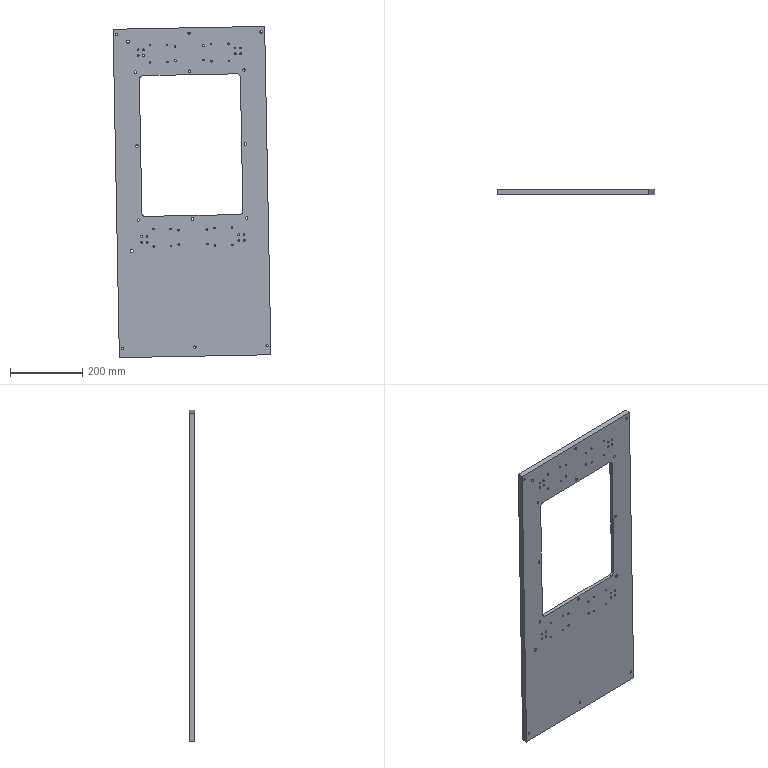Component | SolidWorks | 09Panel2-1 | 1 solid | 224 faces | box 437.25 x 15 x 917.83 mm | volume 3859009 mm3 | cylinder 134 | cone 68 | plane 22 | commonest cylinder face diameters 5 x48 4.2 x32 6.8 x16 11 x12 6.6 x12 8.5 x4 30 x4 20 x4 | material A3 Steel
build123d program:
from build123d import *

# Parameters (mm, degrees)
SKETCH1_W                                          = 900
SKETCH1_H                                          = 420
BOSS_EXTRUDE1_DEPTH                                = 7.5
HOLE_SIZE_ACCORDING_TO_TYPE_1_OF_HEXAG_D           = 6.6
HOLE_SIZE_ACCORDING_TO_TYPE_1_OF_HEXAG_CBORE_D     = 11
HOLE_SIZE_ACCORDING_TO_TYPE_1_OF_HEXAG_CBORE_DEPTH = 8
M10_TAPPED_HOLE1_D                                 = 8.5
M10_TAPPED_HOLE1_CSINK_D                           = 10.05
M10_TAPPED_HOLE1_CSINK_ANGLE                       = 90
CUT_EXTRUDE1_DEPTH                                 = 6
CUT_EXTRUDE2_DEPTH                                 = 497.67
M8_TAPPED_HOLE1_D                                  = 6.8
M8_TAPPED_HOLE1_CSINK_D                            = 8.05
M8_TAPPED_HOLE1_CSINK_ANGLE                        = 90
SKETCH12_R                                         = 20
CUT_EXTRUDE3_DEPTH                                 = 497.815
M6_TAPPED_HOLE1_D                                  = 5
M6_TAPPED_HOLE1_CSINK_D                            = 6.05
M6_TAPPED_HOLE1_CSINK_ANGLE                        = 90
LPATTERN1_COUNT                                    = 2
LPATTERN1_PITCH                                    = 510
M5_TAPPED_HOLE1_D                                  = 4.2
M5_TAPPED_HOLE1_CSINK_D                            = 5.05
M5_TAPPED_HOLE1_CSINK_ANGLE                        = 90
LPATTERN3_COUNT                                    = 2
LPATTERN3_PITCH                                    = 170
LPATTERN3_COUNT_DIR2                               = 2
LPATTERN3_PITCH_DIR2                               = 510
CUT_EXTRUDE4_REACH                                 = 617.594
SKETCH20_R                                         = 6.062
M6_TAPPED_HOLE2_D                                  = 5
MIRROR2_COPY_1_D                                   = 5
SKETCH24_W                                         = 15
SKETCH24_H                                         = 420
BOSS_EXTRUDE2_DEPTH                                = 10
BOSS_EXTRUDE3_START                                = -15
SKETCH25_R                                         = 20
BOSS_EXTRUDE3_DEPTH                                = 15


with BuildPart() as part:
    # Sketch1 → Boss-Extrude1 (new, symmetric)
    with BuildSketch(Plane.XY):
        Rectangle(SKETCH1_W, SKETCH1_H)
    extrude(amount=BOSS_EXTRUDE1_DEPTH, both=True)

    # Hole Size _According to_ Type 1 of Hexag (through all)
    with Locations(Plane(origin=(-435, 200, 7.5), x_dir=(1, 0, 0), z_dir=(0, 0, 1))):
        with Locations((0, 0), (870, 0), (870, -400), (0, -400), (0, -200), (870, -200)):
            CounterBoreHole(HOLE_SIZE_ACCORDING_TO_TYPE_1_OF_HEXAG_D / 2, HOLE_SIZE_ACCORDING_TO_TYPE_1_OF_HEXAG_CBORE_D / 2, HOLE_SIZE_ACCORDING_TO_TYPE_1_OF_HEXAG_CBORE_DEPTH)

    # M10 Tapped Hole1 (through all)
    with Locations(Plane(origin=(-165, -170, 7.5), x_dir=(1, 0, 0), z_dir=(0, 0, 1))):
        with Locations((0, 0), (580, 0)):
            CounterSinkHole(M10_TAPPED_HOLE1_D / 2, M10_TAPPED_HOLE1_CSINK_D / 2, counter_sink_angle=M10_TAPPED_HOLE1_CSINK_ANGLE)

    # Sketch8 → Cut-Extrude1 (cut)
    with BuildSketch(Plane.XY.offset(7.5)):
        with BuildLine():
            Line((-80, -165), (330, -165))
            ThreePointArc((330, -165), (340.607, -160.607), (345, -150))
            Line((345, -150), (345, 150))
            ThreePointArc((345, 150), (340.607, 160.607), (330, 165))
            Line((330, 165), (-80, 165))
            ThreePointArc((-80, 165), (-90.607, 160.607), (-95, 150))
            Line((-95, 150), (-95, -150))
            ThreePointArc((-95, -150), (-90.607, -160.607), (-80, -165))
        make_face()
    extrude(amount=-CUT_EXTRUDE1_DEPTH, mode=Mode.SUBTRACT)

    # Sketch9 → Cut-Extrude2 (cut, through all)
    with BuildSketch(Plane.XY.offset(1.5)):
        with BuildLine():
            Line((-60, -140), (310, -140))
            ThreePointArc((310, -140), (317.071, -137.071), (320, -130))
            Line((320, -130), (320, 130))
            ThreePointArc((320, 130), (317.071, 137.071), (310, 140))
            Line((310, 140), (-60, 140))
            ThreePointArc((-60, 140), (-67.071, 137.071), (-70, 130))
            Line((-70, 130), (-70, -130))
            ThreePointArc((-70, -130), (-67.071, -137.071), (-60, -140))
        make_face()
    extrude(amount=-CUT_EXTRUDE2_DEPTH, mode=Mode.SUBTRACT)

    # M8 Tapped Hole1 (through all)
    with Locations(Plane(origin=(-80, 150, 1.5), x_dir=(1, 0, 0), z_dir=(0, 0, 1))):
        with Locations((0, 0), (410, 0), (410, -300), (0, -300), (0, -150), (205, -300), (205, 0), (410, -150)):
            CounterSinkHole(M8_TAPPED_HOLE1_D / 2, M8_TAPPED_HOLE1_CSINK_D / 2, counter_sink_angle=M8_TAPPED_HOLE1_CSINK_ANGLE)

    # Sketch12 → Cut-Extrude3 (cut, through all)
    with BuildSketch(Plane.XY.offset(7.5)):
        with Locations((-130, 85)):
            Circle(SKETCH12_R)
        with Locations((-130, -85)):
            Circle(SKETCH12_R)
        with Locations((380, 85)):
            Circle(SKETCH12_R)
        with Locations((380, -85)):
            Circle(SKETCH12_R)
    extrude(amount=-CUT_EXTRUDE3_DEPTH, mode=Mode.SUBTRACT)

    # M6 Tapped Hole1 (through all)
    with Locations(Plane(origin=(400, 39.25, 7.5), x_dir=(1, 0, 0), z_dir=(0, 0, 1))):
        with Locations((0, 0), (0, -78.5), (-40, 0), (-40, -78.5)):
            m6_tapped_hole1 = CounterSinkHole(M6_TAPPED_HOLE1_D / 2, M6_TAPPED_HOLE1_CSINK_D / 2, counter_sink_angle=M6_TAPPED_HOLE1_CSINK_ANGLE)

    # LPattern1: M6 Tapped Hole1 ×2
    with Locations(*[(-i * LPATTERN1_PITCH, 0, 0) for i in range(1, LPATTERN1_COUNT)]):
        add(m6_tapped_hole1, mode=Mode.SUBTRACT)

    # M5 Tapped Hole1 (through all)
    with Locations(Plane(origin=(404, -109, 7.5), x_dir=(1, 0, 0), z_dir=(0, 0, 1))):
        with Locations((0, 0), (-48, 0), (-48, 48), (0, 48)):
            m5_tapped_hole1 = CounterSinkHole(M5_TAPPED_HOLE1_D / 2, M5_TAPPED_HOLE1_CSINK_D / 2, counter_sink_angle=M5_TAPPED_HOLE1_CSINK_ANGLE)

    # LPattern3: M5 Tapped Hole1 2 × 2
    with Locations(*[(-j * LPATTERN3_PITCH_DIR2, i * LPATTERN3_PITCH, 0) for i in range(LPATTERN3_COUNT) for j in range(LPATTERN3_COUNT_DIR2) if (i, j) != (0, 0)]):
        add(m5_tapped_hole1, mode=Mode.SUBTRACT)

    # Sketch20 → Cut-Extrude4 (cut, up to next)
    with BuildSketch(Plane(origin=(0, 210, 0), x_dir=(1, 0, 0), z_dir=(0, 1, 0)), mode=Mode.PRIVATE) as cut_extrude4_sk1:
        with Locations((268.5, -11.562)):
            Circle(SKETCH20_R)
    cut_extrude4_tool1 = extrude(cut_extrude4_sk1.sketch, amount=-CUT_EXTRUDE4_REACH, mode=Mode.PRIVATE) & part.part
    # Sketch20 → Cut-Extrude4 (cut, up to next)
    with BuildSketch(Plane(origin=(0, 210, 0), x_dir=(1, 0, 0), z_dir=(0, 1, 0)), mode=Mode.PRIVATE) as cut_extrude4_sk2:
        with Locations((-18.5, -11.562)):
            Circle(SKETCH20_R)
    cut_extrude4_tool2 = extrude(cut_extrude4_sk2.sketch, amount=-CUT_EXTRUDE4_REACH, mode=Mode.PRIVATE) & part.part
    add(cut_extrude4_tool1.solids().sort_by_distance((268.5, 210, 11.562))[0], mode=Mode.SUBTRACT)
    add(cut_extrude4_tool2.solids().sort_by_distance((-18.5, 210, 11.562))[0], mode=Mode.SUBTRACT)

    # M6 Tapped Hole2 (through all)
    with Locations(Plane(origin=(375.5, 127, 7.5), x_dir=(1, 0, 0), z_dir=(0, 0, 1))):
        with Locations((0, 0), (0, 15), (16, 15), (16, 0)):
            m6_tapped_hole2 = Hole(M6_TAPPED_HOLE2_D / 2)

    # Mirror1: M6 Tapped Hole2 across plane
    add(m6_tapped_hole2.mirror(Plane.ZX), mode=Mode.SUBTRACT)

    # Mirror2: M6 Tapped Hole2 across plane
    add(m6_tapped_hole2.mirror(Plane.ZY.offset(-125)), mode=Mode.SUBTRACT)

    # Mirror2 copy 1 (through all)
    with Locations(Plane(origin=(-125.5, -127, 7.5), x_dir=(-1, 0, 0), z_dir=(0, 0, 1))):
        with Locations((0, 0), (0, 15), (16, 15), (16, 0)):
            Hole(MIRROR2_COPY_1_D / 2)

    # Sketch24 → Boss-Extrude2 (add)
    with BuildSketch(Plane.ZY.offset(450)):
        Rectangle(SKETCH24_W, SKETCH24_H)
    extrude(amount=BOSS_EXTRUDE2_DEPTH)

    # Sketch25 → Boss-Extrude3 (add)
    with BuildSketch(Plane(origin=(0, 0, -7.5), x_dir=(-1, 0, 0), z_dir=(0, 0, -1)).offset(BOSS_EXTRUDE3_START)):
        with Locations((-380, 85)):
            Circle(SKETCH25_R)
        with Locations((130, 85)):
            Circle(SKETCH25_R)
        with Locations((-380, -85)):
            Circle(SKETCH25_R)
        with Locations((130, -85)):
            Circle(SKETCH25_R)
    extrude(amount=BOSS_EXTRUDE3_DEPTH)


solid = part.part

# Placed as in the assembly
solid = solid.moved(Location((225.259, -1623.022, 1944.385), (-90, 0, -91.091)))